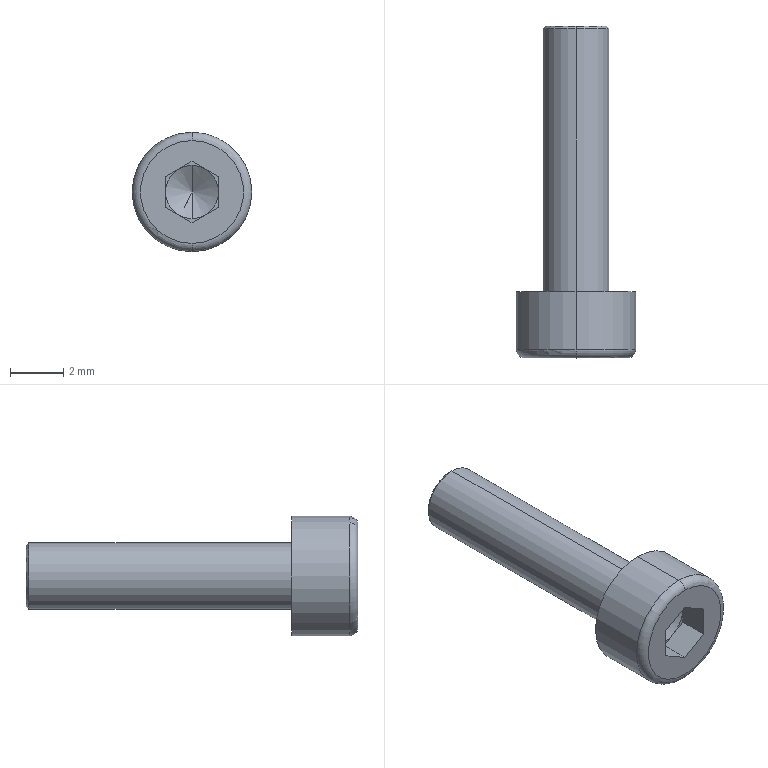Component | SolidWorks | hexagon socket head cap screws gb-10 | 1 solid | 25 faces | box 4.5 x 12.5 x 4.5 mm | volume 84 mm3 | plane 15 | cone 4 | cylinder 4 | torus 2 | commonest cylinder face diameters 2.5 x2 4.5 x2
build123d program:
from build123d import *

# Parameters (mm, degrees)
SKETCH1_R           = 2.25
BASEHEAD_DEPTH      = 2.5
SKETCH2_R           = 1.25
BASEBODY_DEPTH      = 10
HEXAGONSOCKET_DEPTH = 1.1
TOPFILLET_R         = 0.3125
CHAMFER1_SIZE       = 0.1


with BuildPart() as part:
    # Sketch1 → BaseHead (new body)
    with BuildSketch(Plane(origin=(0, 0, 0), x_dir=(0, 0, -1), z_dir=(1, 0, 0))):
        Circle(SKETCH1_R)
    extrude(amount=BASEHEAD_DEPTH)

    # Sketch2 → BaseBody (add)
    with BuildSketch(Plane(origin=(2.5, 0, 0), x_dir=(0, 0, -1), z_dir=(1, 0, 0))):
        Circle(SKETCH2_R)
    extrude(amount=BASEBODY_DEPTH)

    # Sketch3 → HexagonSocket (cut)
    with BuildSketch(Plane(origin=(0, 0, 0), x_dir=(0, 0, -1), z_dir=(1, 0, 0))):
        Polygon((1.155, 0), (0.5774, 1), (-0.5774, 1), (-1.155, 0), (-0.5774, -1), (0.5774, -1), align=None)
    extrude(amount=HEXAGONSOCKET_DEPTH, mode=Mode.SUBTRACT)

    # Sketch4 → Cut-Revolve1 (revolve, cut)
    with BuildSketch(Plane(origin=(-4.196, 0.75, 0), x_dir=(-1, 0, 0), z_dir=(0, 0, 1)), mode=Mode.PRIVATE) as cut_revolve1_sk:
        Polygon((-5.296, 1.75), (-5.873, 0.75), (-5.296, 0.75), align=None)
    revolve(cut_revolve1_sk.sketch.rotate(Axis((0.839, 0, 0), (-1, 0, 0)), 90), axis=Axis((0.839, 0, 0), (-1, 0, 0)), mode=Mode.SUBTRACT)

    # TopFillet
    topfillet_edges = [part.edges().sort_by_distance(p)[0] for p in [
        (0, 0, 2.25),
    ]]
    fillet(topfillet_edges, radius=TOPFILLET_R)

    # Chamfer1
    chamfer1_edges = [part.edges().sort_by_distance(p)[0] for p in [
        (12.5, 0, 1.25),
    ]]
    chamfer(chamfer1_edges, length=CHAMFER1_SIZE)


solid = part.part

# Placed as in the assembly
solid = solid.moved(Location((51.034, -16.994, 238.475), (0, 0, 90)))
STEP:
#1=CARTESIAN_POINT('',(2.009,-0.1769,9.343));
#2=VERTEX_POINT('',#1);
#3=CARTESIAN_POINT('',(2.009,-0.1769,9.434));
#4=VERTEX_POINT('',#3);
#5=CARTESIAN_POINT('',(2.009,-0.1769,9.389));
#6=DIRECTION('',(0.,1.,0.));
#7=DIRECTION('',(0.,0.,-1.));
#8=AXIS2_PLACEMENT_3D('',#5,#6,#7);
#9=CIRCLE('',#8,0.04528);
#10=EDGE_CURVE('',#2,#4,#9,.T.);
#11=ORIENTED_EDGE('',*,*,#10,.F.);
#12=CARTESIAN_POINT('',(2.009,-0.1809,9.34));
#13=VERTEX_POINT('',#12);
#14=CARTESIAN_POINT('',(2.009,-0.1769,9.343));
#15=DIRECTION('',(-0.,-0.7071,-0.7071));
#16=VECTOR('',#15,39.37);
#17=LINE('',#14,#16);
#18=EDGE_CURVE('',#2,#13,#17,.T.);
#19=ORIENTED_EDGE('',*,*,#18,.T.);
#20=CARTESIAN_POINT('',(2.009,-0.1809,9.438));
#21=VERTEX_POINT('',#20);
#22=CARTESIAN_POINT('',(2.009,-0.1809,9.389));
#23=DIRECTION('',(0.,-1.,0.));
#24=DIRECTION('',(0.,0.,-1.));
#25=AXIS2_PLACEMENT_3D('',#22,#23,#24);
#26=CIRCLE('',#25,0.04921);
#27=EDGE_CURVE('',#21,#13,#26,.T.);
#28=ORIENTED_EDGE('',*,*,#27,.F.);
#29=CARTESIAN_POINT('',(2.009,-0.1769,9.434));
#30=DIRECTION('',(0.,-0.7071,0.7071));
#31=VECTOR('',#30,39.37);
#32=LINE('',#29,#31);
#33=EDGE_CURVE('',#4,#21,#32,.T.);
#34=ORIENTED_EDGE('',*,*,#33,.F.);
#35=EDGE_LOOP('',(#11,#19,#28,#34));
#36=FACE_OUTER_BOUND('',#35,.T.);
#37=CARTESIAN_POINT('',(2.009,-0.1769,9.389));
#38=DIRECTION('',(0.,-1.,0.));
#39=DIRECTION('',(0.,0.,1.));
#40=AXIS2_PLACEMENT_3D('',#37,#38,#39);
#41=CONICAL_SURFACE('',#40,0.04528,0.7854);
#42=ADVANCED_FACE('',(#36),#41,.T.);
#43=CARTESIAN_POINT('',(2.009,-0.669,9.465));
#44=VERTEX_POINT('',#43);
#45=CARTESIAN_POINT('',(2.009,-0.669,9.312));
#46=VERTEX_POINT('',#45);
#47=CARTESIAN_POINT('',(2.009,-0.669,9.389));
#48=DIRECTION('',(0.,-1.,0.));
#49=DIRECTION('',(0.,0.,-1.));
#50=AXIS2_PLACEMENT_3D('',#47,#48,#49);
#51=CIRCLE('',#50,0.07628);
#52=EDGE_CURVE('',#44,#46,#51,.T.);
#53=ORIENTED_EDGE('',*,*,#52,.F.);
#54=CARTESIAN_POINT('',(2.009,-0.6567,9.477));
#55=VERTEX_POINT('',#54);
#56=CARTESIAN_POINT('',(2.009,-0.6567,9.465));
#57=DIRECTION('',(-1.,0.,-0.));
#58=DIRECTION('',(0.,0.,1.));
#59=AXIS2_PLACEMENT_3D('',#56,#57,#58);
#60=CIRCLE('',#59,0.0123);
#61=EDGE_CURVE('',#44,#55,#60,.T.);
#62=ORIENTED_EDGE('',*,*,#61,.T.);
#63=CARTESIAN_POINT('',(2.009,-0.6567,9.3));
#64=VERTEX_POINT('',#63);
#65=CARTESIAN_POINT('',(2.009,-0.6567,9.389));
#66=DIRECTION('',(0.,1.,0.));
#67=DIRECTION('',(0.,0.,-1.));
#68=AXIS2_PLACEMENT_3D('',#65,#66,#67);
#69=CIRCLE('',#68,0.08858);
#70=EDGE_CURVE('',#64,#55,#69,.T.);
#71=ORIENTED_EDGE('',*,*,#70,.F.);
#72=CARTESIAN_POINT('',(2.009,-0.6567,9.312));
#73=DIRECTION('',(1.,0.,0.));
#74=DIRECTION('',(0.,0.,-1.));
#75=AXIS2_PLACEMENT_3D('',#72,#73,#74);
#76=CIRCLE('',#75,0.0123);
#77=EDGE_CURVE('',#46,#64,#76,.T.);
#78=ORIENTED_EDGE('',*,*,#77,.F.);
#79=EDGE_LOOP('',(#53,#62,#71,#78));
#80=FACE_OUTER_BOUND('',#79,.T.);
#81=CARTESIAN_POINT('',(2.009,-0.6567,9.389));
#82=DIRECTION('',(0.,1.,0.));
#83=DIRECTION('',(0.,0.,-1.));
#84=AXIS2_PLACEMENT_3D('',#81,#82,#83);
#85=TOROIDAL_SURFACE('',#84,0.07628,0.0123);
#86=ADVANCED_FACE('',(#80),#85,.T.);
#87=CARTESIAN_POINT('',(2.009,-0.603,9.389));
#88=VERTEX_POINT('',#87);
#89=CARTESIAN_POINT('',(2.009,-0.6257,9.428));
#90=VERTEX_POINT('',#89);
#91=CARTESIAN_POINT('',(2.009,-0.6257,9.428));
#92=DIRECTION('',(0.,-0.5,0.866));
#93=VECTOR('',#92,39.37);
#94=LINE('',#91,#93);
#95=EDGE_CURVE('',#88,#90,#94,.T.);
#96=ORIENTED_EDGE('',*,*,#95,.F.);
#97=CARTESIAN_POINT('',(2.009,-0.6257,9.349));
#98=VERTEX_POINT('',#97);
#99=CARTESIAN_POINT('',(2.009,-0.6257,9.349));
#100=DIRECTION('',(-0.,-0.5,-0.866));
#101=VECTOR('',#100,39.37);
#102=LINE('',#99,#101);
#103=EDGE_CURVE('',#88,#98,#102,.T.);
#104=ORIENTED_EDGE('',*,*,#103,.T.);
#105=CARTESIAN_POINT('',(2.029,-0.6257,9.355));
#106=VERTEX_POINT('',#105);
#107=CARTESIAN_POINT('',(2.009,-0.6257,9.389));
#108=DIRECTION('',(0.,-1.,0.));
#109=DIRECTION('',(0.,0.,-1.));
#110=AXIS2_PLACEMENT_3D('',#107,#108,#109);
#111=CIRCLE('',#110,0.03937);
#112=EDGE_CURVE('',#98,#106,#111,.T.);
#113=ORIENTED_EDGE('',*,*,#112,.T.);
#114=CARTESIAN_POINT('',(2.049,-0.6257,9.389));
#115=VERTEX_POINT('',#114);
#116=CARTESIAN_POINT('',(2.009,-0.6257,9.389));
#117=DIRECTION('',(0.,-1.,0.));
#118=DIRECTION('',(0.,0.,-1.));
#119=AXIS2_PLACEMENT_3D('',#116,#117,#118);
#120=CIRCLE('',#119,0.03937);
#121=EDGE_CURVE('',#106,#115,#120,.T.);
#122=ORIENTED_EDGE('',*,*,#121,.T.);
#123=CARTESIAN_POINT('',(2.029,-0.6257,9.423));
#124=VERTEX_POINT('',#123);
#125=CARTESIAN_POINT('',(2.009,-0.6257,9.389));
#126=DIRECTION('',(0.,-1.,0.));
#127=DIRECTION('',(0.,0.,-1.));
#128=AXIS2_PLACEMENT_3D('',#125,#126,#127);
#129=CIRCLE('',#128,0.03937);
#130=EDGE_CURVE('',#115,#124,#129,.T.);
#131=ORIENTED_EDGE('',*,*,#130,.T.);
#132=CARTESIAN_POINT('',(2.009,-0.6257,9.389));
#133=DIRECTION('',(0.,-1.,0.));
#134=DIRECTION('',(0.,0.,-1.));
#135=AXIS2_PLACEMENT_3D('',#132,#133,#134);
#136=CIRCLE('',#135,0.03937);
#137=EDGE_CURVE('',#124,#90,#136,.T.);
#138=ORIENTED_EDGE('',*,*,#137,.T.);
#139=EDGE_LOOP('',(#96,#104,#113,#122,#131,#138));
#140=FACE_OUTER_BOUND('',#139,.T.);
#141=CARTESIAN_POINT('',(2.009,-0.6257,9.389));
#142=DIRECTION('',(0.,-1.,0.));
#143=DIRECTION('',(0.,0.,1.));
#144=AXIS2_PLACEMENT_3D('',#141,#142,#143);
#145=CONICAL_SURFACE('',#144,0.03937,1.047);
#146=ADVANCED_FACE('',(#140),#145,.F.);
#147=ORIENTED_EDGE('',*,*,#27,.T.);
#148=CARTESIAN_POINT('',(2.009,-0.5706,9.34));
#149=VERTEX_POINT('',#148);
#150=CARTESIAN_POINT('',(2.009,-0.1769,9.34));
#151=DIRECTION('',(0.,-1.,0.));
#152=VECTOR('',#151,39.37);
#153=LINE('',#150,#152);
#154=EDGE_CURVE('',#13,#149,#153,.T.);
#155=ORIENTED_EDGE('',*,*,#154,.T.);
#156=CARTESIAN_POINT('',(2.009,-0.5706,9.438));
#157=VERTEX_POINT('',#156);
#158=CARTESIAN_POINT('',(2.009,-0.5706,9.389));
#159=DIRECTION('',(0.,1.,0.));
#160=DIRECTION('',(0.,0.,-1.));
#161=AXIS2_PLACEMENT_3D('',#158,#159,#160);
#162=CIRCLE('',#161,0.04921);
#163=EDGE_CURVE('',#149,#157,#162,.T.);
#164=ORIENTED_EDGE('',*,*,#163,.T.);
#165=CARTESIAN_POINT('',(2.009,-0.1769,9.438));
#166=DIRECTION('',(0.,-1.,0.));
#167=VECTOR('',#166,39.37);
#168=LINE('',#165,#167);
#169=EDGE_CURVE('',#21,#157,#168,.T.);
#170=ORIENTED_EDGE('',*,*,#169,.F.);
#171=EDGE_LOOP('',(#147,#155,#164,#170));
#172=FACE_OUTER_BOUND('',#171,.T.);
#173=CARTESIAN_POINT('',(2.009,-0.1769,9.389));
#174=DIRECTION('',(0.,-1.,0.));
#175=DIRECTION('',(0.,0.,1.));
#176=AXIS2_PLACEMENT_3D('',#173,#174,#175);
#177=CYLINDRICAL_SURFACE('',#176,0.04921);
#178=ADVANCED_FACE('',(#172),#177,.T.);
#179=CARTESIAN_POINT('',(2.009,-0.5706,9.3));
#180=VERTEX_POINT('',#179);
#181=CARTESIAN_POINT('',(2.009,-0.5706,9.477));
#182=VERTEX_POINT('',#181);
#183=CARTESIAN_POINT('',(2.009,-0.5706,9.389));
#184=DIRECTION('',(0.,1.,0.));
#185=DIRECTION('',(0.,0.,-1.));
#186=AXIS2_PLACEMENT_3D('',#183,#184,#185);
#187=CIRCLE('',#186,0.08858);
#188=EDGE_CURVE('',#180,#182,#187,.T.);
#189=ORIENTED_EDGE('',*,*,#188,.F.);
#190=CARTESIAN_POINT('',(2.009,-0.5706,9.3));
#191=DIRECTION('',(0.,-1.,0.));
#192=VECTOR('',#191,39.37);
#193=LINE('',#190,#192);
#194=EDGE_CURVE('',#180,#64,#193,.T.);
#195=ORIENTED_EDGE('',*,*,#194,.T.);
#196=ORIENTED_EDGE('',*,*,#70,.T.);
#197=CARTESIAN_POINT('',(2.009,-0.5706,9.477));
#198=DIRECTION('',(0.,-1.,0.));
#199=VECTOR('',#198,39.37);
#200=LINE('',#197,#199);
#201=EDGE_CURVE('',#182,#55,#200,.T.);
#202=ORIENTED_EDGE('',*,*,#201,.F.);
#203=EDGE_LOOP('',(#189,#195,#196,#202));
#204=FACE_OUTER_BOUND('',#203,.T.);
#205=CARTESIAN_POINT('',(2.009,-0.5706,9.389));
#206=DIRECTION('',(0.,-1.,0.));
#207=DIRECTION('',(0.,0.,1.));
#208=AXIS2_PLACEMENT_3D('',#205,#206,#207);
#209=CYLINDRICAL_SURFACE('',#208,0.08858);
#210=ADVANCED_FACE('',(#204),#209,.T.);
#211=ORIENTED_EDGE('',*,*,#121,.F.);
#212=CARTESIAN_POINT('',(2.049,-0.6257,9.366));
#213=VERTEX_POINT('',#212);
#214=CARTESIAN_POINT('',(2.049,-0.6257,9.366));
#215=DIRECTION('',(-0.866,0.,-0.5));
#216=VECTOR('',#215,39.37);
#217=LINE('',#214,#216);
#218=EDGE_CURVE('',#213,#106,#217,.T.);
#219=ORIENTED_EDGE('',*,*,#218,.F.);
#220=CARTESIAN_POINT('',(2.049,-0.6257,9.411));
#221=DIRECTION('',(-0.,0.,-1.));
#222=VECTOR('',#221,39.37);
#223=LINE('',#220,#222);
#224=EDGE_CURVE('',#115,#213,#223,.T.);
#225=ORIENTED_EDGE('',*,*,#224,.F.);
#226=EDGE_LOOP('',(#211,#219,#225));
#227=FACE_OUTER_BOUND('',#226,.T.);
#228=CARTESIAN_POINT('',(2.009,-0.6257,9.343));
#229=DIRECTION('',(0.,1.,0.));
#230=DIRECTION('',(0.,0.,-1.));
#231=AXIS2_PLACEMENT_3D('',#228,#229,#230);
#232=PLANE('',#231);
#233=ADVANCED_FACE('',(#227),#232,.F.);
#234=ORIENTED_EDGE('',*,*,#130,.F.);
#235=CARTESIAN_POINT('',(2.049,-0.6257,9.411));
#236=VERTEX_POINT('',#235);
#237=CARTESIAN_POINT('',(2.049,-0.6257,9.411));
#238=DIRECTION('',(-0.,0.,-1.));
#239=VECTOR('',#238,39.37);
#240=LINE('',#237,#239);
#241=EDGE_CURVE('',#236,#115,#240,.T.);
#242=ORIENTED_EDGE('',*,*,#241,.F.);
#243=CARTESIAN_POINT('',(2.009,-0.6257,9.434));
#244=DIRECTION('',(0.866,0.,-0.5));
#245=VECTOR('',#244,39.37);
#246=LINE('',#243,#245);
#247=EDGE_CURVE('',#124,#236,#246,.T.);
#248=ORIENTED_EDGE('',*,*,#247,.F.);
#249=EDGE_LOOP('',(#234,#242,#248));
#250=FACE_OUTER_BOUND('',#249,.T.);
#251=CARTESIAN_POINT('',(2.009,-0.6257,9.343));
#252=DIRECTION('',(0.,1.,0.));
#253=DIRECTION('',(0.,0.,-1.));
#254=AXIS2_PLACEMENT_3D('',#251,#252,#253);
#255=PLANE('',#254);
#256=ADVANCED_FACE('',(#250),#255,.F.);
#257=ORIENTED_EDGE('',*,*,#137,.F.);
#258=CARTESIAN_POINT('',(2.009,-0.6257,9.434));
#259=VERTEX_POINT('',#258);
#260=CARTESIAN_POINT('',(2.009,-0.6257,9.434));
#261=DIRECTION('',(0.866,0.,-0.5));
#262=VECTOR('',#261,39.37);
#263=LINE('',#260,#262);
#264=EDGE_CURVE('',#259,#124,#263,.T.);
#265=ORIENTED_EDGE('',*,*,#264,.F.);
#266=CARTESIAN_POINT('',(1.99,-0.6257,9.423));
#267=VERTEX_POINT('',#266);
#268=CARTESIAN_POINT('',(1.97,-0.6257,9.411));
#269=DIRECTION('',(0.866,0.,0.5));
#270=VECTOR('',#269,39.37);
#271=LINE('',#268,#270);
#272=EDGE_CURVE('',#267,#259,#271,.T.);
#273=ORIENTED_EDGE('',*,*,#272,.F.);
#274=CARTESIAN_POINT('',(2.009,-0.6257,9.389));
#275=DIRECTION('',(0.,-1.,0.));
#276=DIRECTION('',(0.,0.,-1.));
#277=AXIS2_PLACEMENT_3D('',#274,#275,#276);
#278=CIRCLE('',#277,0.03937);
#279=EDGE_CURVE('',#90,#267,#278,.T.);
#280=ORIENTED_EDGE('',*,*,#279,.F.);
#281=EDGE_LOOP('',(#257,#265,#273,#280));
#282=FACE_OUTER_BOUND('',#281,.T.);
#283=CARTESIAN_POINT('',(2.009,-0.6257,9.343));
#284=DIRECTION('',(0.,1.,0.));
#285=DIRECTION('',(0.,0.,-1.));
#286=AXIS2_PLACEMENT_3D('',#283,#284,#285);
#287=PLANE('',#286);
#288=ADVANCED_FACE('',(#282),#287,.F.);
#289=CARTESIAN_POINT('',(1.97,-0.6257,9.389));
#290=VERTEX_POINT('',#289);
#291=CARTESIAN_POINT('',(2.009,-0.6257,9.389));
#292=DIRECTION('',(0.,-1.,0.));
#293=DIRECTION('',(0.,0.,-1.));
#294=AXIS2_PLACEMENT_3D('',#291,#292,#293);
#295=CIRCLE('',#294,0.03937);
#296=EDGE_CURVE('',#267,#290,#295,.T.);
#297=ORIENTED_EDGE('',*,*,#296,.F.);
#298=CARTESIAN_POINT('',(1.97,-0.6257,9.411));
#299=VERTEX_POINT('',#298);
#300=CARTESIAN_POINT('',(1.97,-0.6257,9.411));
#301=DIRECTION('',(0.866,0.,0.5));
#302=VECTOR('',#301,39.37);
#303=LINE('',#300,#302);
#304=EDGE_CURVE('',#299,#267,#303,.T.);
#305=ORIENTED_EDGE('',*,*,#304,.F.);
#306=CARTESIAN_POINT('',(1.97,-0.6257,9.366));
#307=DIRECTION('',(0.,0.,1.));
#308=VECTOR('',#307,39.37);
#309=LINE('',#306,#308);
#310=EDGE_CURVE('',#290,#299,#309,.T.);
#311=ORIENTED_EDGE('',*,*,#310,.F.);
#312=EDGE_LOOP('',(#297,#305,#311));
#313=FACE_OUTER_BOUND('',#312,.T.);
#314=CARTESIAN_POINT('',(2.009,-0.6257,9.343));
#315=DIRECTION('',(0.,1.,0.));
#316=DIRECTION('',(0.,0.,-1.));
#317=AXIS2_PLACEMENT_3D('',#314,#315,#316);
#318=PLANE('',#317);
#319=ADVANCED_FACE('',(#313),#318,.F.);
#320=CARTESIAN_POINT('',(1.99,-0.6257,9.355));
#321=VERTEX_POINT('',#320);
#322=CARTESIAN_POINT('',(2.009,-0.6257,9.389));
#323=DIRECTION('',(0.,1.,0.));
#324=DIRECTION('',(0.,0.,-1.));
#325=AXIS2_PLACEMENT_3D('',#322,#323,#324);
#326=CIRCLE('',#325,0.03937);
#327=EDGE_CURVE('',#321,#290,#326,.T.);
#328=ORIENTED_EDGE('',*,*,#327,.T.);
#329=CARTESIAN_POINT('',(1.97,-0.6257,9.366));
#330=VERTEX_POINT('',#329);
#331=CARTESIAN_POINT('',(1.97,-0.6257,9.366));
#332=DIRECTION('',(0.,0.,1.));
#333=VECTOR('',#332,39.37);
#334=LINE('',#331,#333);
#335=EDGE_CURVE('',#330,#290,#334,.T.);
#336=ORIENTED_EDGE('',*,*,#335,.F.);
#337=CARTESIAN_POINT('',(2.009,-0.6257,9.343));
#338=DIRECTION('',(-0.866,0.,0.5));
#339=VECTOR('',#338,39.37);
#340=LINE('',#337,#339);
#341=EDGE_CURVE('',#321,#330,#340,.T.);
#342=ORIENTED_EDGE('',*,*,#341,.F.);
#343=EDGE_LOOP('',(#328,#336,#342));
#344=FACE_OUTER_BOUND('',#343,.T.);
#345=CARTESIAN_POINT('',(2.009,-0.6257,9.343));
#346=DIRECTION('',(0.,1.,0.));
#347=DIRECTION('',(0.,0.,-1.));
#348=AXIS2_PLACEMENT_3D('',#345,#346,#347);
#349=PLANE('',#348);
#350=ADVANCED_FACE('',(#344),#349,.F.);
#351=CARTESIAN_POINT('',(2.009,-0.6257,9.389));
#352=DIRECTION('',(0.,-1.,0.));
#353=DIRECTION('',(0.,0.,-1.));
#354=AXIS2_PLACEMENT_3D('',#351,#352,#353);
#355=CIRCLE('',#354,0.03937);
#356=EDGE_CURVE('',#321,#98,#355,.T.);
#357=ORIENTED_EDGE('',*,*,#356,.F.);
#358=CARTESIAN_POINT('',(2.009,-0.6257,9.343));
#359=VERTEX_POINT('',#358);
#360=CARTESIAN_POINT('',(2.009,-0.6257,9.343));
#361=DIRECTION('',(-0.866,0.,0.5));
#362=VECTOR('',#361,39.37);
#363=LINE('',#360,#362);
#364=EDGE_CURVE('',#359,#321,#363,.T.);
#365=ORIENTED_EDGE('',*,*,#364,.F.);
#366=CARTESIAN_POINT('',(2.049,-0.6257,9.366));
#367=DIRECTION('',(-0.866,0.,-0.5));
#368=VECTOR('',#367,39.37);
#369=LINE('',#366,#368);
#370=EDGE_CURVE('',#106,#359,#369,.T.);
#371=ORIENTED_EDGE('',*,*,#370,.F.);
#372=ORIENTED_EDGE('',*,*,#112,.F.);
#373=EDGE_LOOP('',(#357,#365,#371,#372));
#374=FACE_OUTER_BOUND('',#373,.T.);
#375=CARTESIAN_POINT('',(2.009,-0.6257,9.343));
#376=DIRECTION('',(0.,1.,0.));
#377=DIRECTION('',(0.,0.,-1.));
#378=AXIS2_PLACEMENT_3D('',#375,#376,#377);
#379=PLANE('',#378);
#380=ADVANCED_FACE('',(#374),#379,.F.);
#381=CARTESIAN_POINT('',(2.009,-0.669,9.389));
#382=DIRECTION('',(0.,-1.,0.));
#383=DIRECTION('',(0.,0.,-1.));
#384=AXIS2_PLACEMENT_3D('',#381,#382,#383);
#385=CIRCLE('',#384,0.07628);
#386=EDGE_CURVE('',#46,#44,#385,.T.);
#387=ORIENTED_EDGE('',*,*,#386,.T.);
#388=ORIENTED_EDGE('',*,*,#52,.T.);
#389=EDGE_LOOP('',(#387,#388));
#390=FACE_OUTER_BOUND('',#389,.T.);
#391=CARTESIAN_POINT('',(2.049,-0.669,9.366));
#392=VERTEX_POINT('',#391);
#393=CARTESIAN_POINT('',(2.009,-0.669,9.343));
#394=VERTEX_POINT('',#393);
#395=CARTESIAN_POINT('',(2.049,-0.669,9.366));
#396=DIRECTION('',(-0.866,0.,-0.5));
#397=VECTOR('',#396,39.37);
#398=LINE('',#395,#397);
#399=EDGE_CURVE('',#392,#394,#398,.T.);
#400=ORIENTED_EDGE('',*,*,#399,.T.);
#401=CARTESIAN_POINT('',(1.97,-0.669,9.366));
#402=VERTEX_POINT('',#401);
#403=CARTESIAN_POINT('',(2.009,-0.669,9.343));
#404=DIRECTION('',(-0.866,0.,0.5));
#405=VECTOR('',#404,39.37);
#406=LINE('',#403,#405);
#407=EDGE_CURVE('',#394,#402,#406,.T.);
#408=ORIENTED_EDGE('',*,*,#407,.T.);
#409=CARTESIAN_POINT('',(1.97,-0.669,9.411));
#410=VERTEX_POINT('',#409);
#411=CARTESIAN_POINT('',(1.97,-0.669,9.366));
#412=DIRECTION('',(0.,0.,1.));
#413=VECTOR('',#412,39.37);
#414=LINE('',#411,#413);
#415=EDGE_CURVE('',#402,#410,#414,.T.);
#416=ORIENTED_EDGE('',*,*,#415,.T.);
#417=CARTESIAN_POINT('',(2.009,-0.669,9.434));
#418=VERTEX_POINT('',#417);
#419=CARTESIAN_POINT('',(1.97,-0.669,9.411));
#420=DIRECTION('',(0.866,0.,0.5));
#421=VECTOR('',#420,39.37);
#422=LINE('',#419,#421);
#423=EDGE_CURVE('',#410,#418,#422,.T.);
#424=ORIENTED_EDGE('',*,*,#423,.T.);
#425=CARTESIAN_POINT('',(2.049,-0.669,9.411));
#426=VERTEX_POINT('',#425);
#427=CARTESIAN_POINT('',(2.009,-0.669,9.434));
#428=DIRECTION('',(0.866,0.,-0.5));
#429=VECTOR('',#428,39.37);
#430=LINE('',#427,#429);
#431=EDGE_CURVE('',#418,#426,#430,.T.);
#432=ORIENTED_EDGE('',*,*,#431,.T.);
#433=CARTESIAN_POINT('',(2.049,-0.669,9.411));
#434=DIRECTION('',(-0.,0.,-1.));
#435=VECTOR('',#434,39.37);
#436=LINE('',#433,#435);
#437=EDGE_CURVE('',#426,#392,#436,.T.);
#438=ORIENTED_EDGE('',*,*,#437,.T.);
#439=EDGE_LOOP('',(#400,#408,#416,#424,#432,#438));
#440=FACE_BOUND('',#439,.T.);
#441=CARTESIAN_POINT('',(2.009,-0.669,9.389));
#442=DIRECTION('',(0.,1.,0.));
#443=DIRECTION('',(0.,0.,-1.));
#444=AXIS2_PLACEMENT_3D('',#441,#442,#443);
#445=PLANE('',#444);
#446=ADVANCED_FACE('',(#390,#440),#445,.F.);
#447=CARTESIAN_POINT('',(2.009,-0.5706,9.389));
#448=DIRECTION('',(0.,1.,0.));
#449=DIRECTION('',(0.,0.,-1.));
#450=AXIS2_PLACEMENT_3D('',#447,#448,#449);
#451=CIRCLE('',#450,0.08858);
#452=EDGE_CURVE('',#182,#180,#451,.T.);
#453=ORIENTED_EDGE('',*,*,#452,.T.);
#454=ORIENTED_EDGE('',*,*,#188,.T.);
#455=EDGE_LOOP('',(#453,#454));
#456=FACE_OUTER_BOUND('',#455,.T.);
#457=CARTESIAN_POINT('',(2.009,-0.5706,9.389));
#458=DIRECTION('',(0.,1.,0.));
#459=DIRECTION('',(0.,0.,-1.));
#460=AXIS2_PLACEMENT_3D('',#457,#458,#459);
#461=CIRCLE('',#460,0.04921);
#462=EDGE_CURVE('',#157,#149,#461,.T.);
#463=ORIENTED_EDGE('',*,*,#462,.F.);
#464=ORIENTED_EDGE('',*,*,#163,.F.);
#465=EDGE_LOOP('',(#463,#464));
#466=FACE_BOUND('',#465,.T.);
#467=CARTESIAN_POINT('',(2.009,-0.5706,9.389));
#468=DIRECTION('',(0.,1.,0.));
#469=DIRECTION('',(0.,0.,-1.));
#470=AXIS2_PLACEMENT_3D('',#467,#468,#469);
#471=PLANE('',#470);
#472=ADVANCED_FACE('',(#456,#466),#471,.T.);
#473=ORIENTED_EDGE('',*,*,#194,.F.);
#474=ORIENTED_EDGE('',*,*,#452,.F.);
#475=ORIENTED_EDGE('',*,*,#201,.T.);
#476=CARTESIAN_POINT('',(2.009,-0.6567,9.389));
#477=DIRECTION('',(0.,1.,0.));
#478=DIRECTION('',(0.,0.,-1.));
#479=AXIS2_PLACEMENT_3D('',#476,#477,#478);
#480=CIRCLE('',#479,0.08858);
#481=EDGE_CURVE('',#55,#64,#480,.T.);
#482=ORIENTED_EDGE('',*,*,#481,.T.);
#483=EDGE_LOOP('',(#473,#474,#475,#482));
#484=FACE_OUTER_BOUND('',#483,.T.);
#485=CARTESIAN_POINT('',(2.009,-0.5706,9.389));
#486=DIRECTION('',(0.,-1.,0.));
#487=DIRECTION('',(0.,0.,1.));
#488=AXIS2_PLACEMENT_3D('',#485,#486,#487);
#489=CYLINDRICAL_SURFACE('',#488,0.08858);
#490=ADVANCED_FACE('',(#484),#489,.T.);
#491=ORIENTED_EDGE('',*,*,#154,.F.);
#492=CARTESIAN_POINT('',(2.009,-0.1809,9.389));
#493=DIRECTION('',(0.,-1.,0.));
#494=DIRECTION('',(0.,0.,-1.));
#495=AXIS2_PLACEMENT_3D('',#492,#493,#494);
#496=CIRCLE('',#495,0.04921);
#497=EDGE_CURVE('',#13,#21,#496,.T.);
#498=ORIENTED_EDGE('',*,*,#497,.T.);
#499=ORIENTED_EDGE('',*,*,#169,.T.);
#500=ORIENTED_EDGE('',*,*,#462,.T.);
#501=EDGE_LOOP('',(#491,#498,#499,#500));
#502=FACE_OUTER_BOUND('',#501,.T.);
#503=CARTESIAN_POINT('',(2.009,-0.1769,9.389));
#504=DIRECTION('',(0.,-1.,0.));
#505=DIRECTION('',(0.,0.,1.));
#506=AXIS2_PLACEMENT_3D('',#503,#504,#505);
#507=CYLINDRICAL_SURFACE('',#506,0.04921);
#508=ADVANCED_FACE('',(#502),#507,.T.);
#509=CARTESIAN_POINT('',(2.009,-0.1769,9.389));
#510=DIRECTION('',(0.,1.,0.));
#511=DIRECTION('',(0.,0.,-1.));
#512=AXIS2_PLACEMENT_3D('',#509,#510,#511);
#513=CIRCLE('',#512,0.04528);
#514=EDGE_CURVE('',#4,#2,#513,.T.);
#515=ORIENTED_EDGE('',*,*,#514,.T.);
#516=ORIENTED_EDGE('',*,*,#10,.T.);
#517=EDGE_LOOP('',(#515,#516));
#518=FACE_OUTER_BOUND('',#517,.T.);
#519=CARTESIAN_POINT('',(2.009,-0.1769,9.389));
#520=DIRECTION('',(0.,1.,0.));
#521=DIRECTION('',(0.,0.,-1.));
#522=AXIS2_PLACEMENT_3D('',#519,#520,#521);
#523=PLANE('',#522);
#524=ADVANCED_FACE('',(#518),#523,.T.);
#525=ORIENTED_EDGE('',*,*,#399,.F.);
#526=CARTESIAN_POINT('',(2.049,-0.6257,9.366));
#527=DIRECTION('',(0.,-1.,0.));
#528=VECTOR('',#527,39.37);
#529=LINE('',#526,#528);
#530=EDGE_CURVE('',#213,#392,#529,.T.);
#531=ORIENTED_EDGE('',*,*,#530,.F.);
#532=ORIENTED_EDGE('',*,*,#218,.T.);
#533=ORIENTED_EDGE('',*,*,#370,.T.);
#534=CARTESIAN_POINT('',(2.009,-0.6257,9.343));
#535=DIRECTION('',(0.,-1.,0.));
#536=VECTOR('',#535,39.37);
#537=LINE('',#534,#536);
#538=EDGE_CURVE('',#359,#394,#537,.T.);
#539=ORIENTED_EDGE('',*,*,#538,.T.);
#540=EDGE_LOOP('',(#525,#531,#532,#533,#539));
#541=FACE_OUTER_BOUND('',#540,.T.);
#542=CARTESIAN_POINT('',(2.049,-0.6257,9.366));
#543=DIRECTION('',(-0.5,0.,0.866));
#544=DIRECTION('',(0.866,0.,0.5));
#545=AXIS2_PLACEMENT_3D('',#542,#543,#544);
#546=PLANE('',#545);
#547=ADVANCED_FACE('',(#541),#546,.T.);
#548=ORIENTED_EDGE('',*,*,#407,.F.);
#549=ORIENTED_EDGE('',*,*,#538,.F.);
#550=ORIENTED_EDGE('',*,*,#364,.T.);
#551=ORIENTED_EDGE('',*,*,#341,.T.);
#552=CARTESIAN_POINT('',(1.97,-0.6257,9.366));
#553=DIRECTION('',(0.,-1.,0.));
#554=VECTOR('',#553,39.37);
#555=LINE('',#552,#554);
#556=EDGE_CURVE('',#330,#402,#555,.T.);
#557=ORIENTED_EDGE('',*,*,#556,.T.);
#558=EDGE_LOOP('',(#548,#549,#550,#551,#557));
#559=FACE_OUTER_BOUND('',#558,.T.);
#560=CARTESIAN_POINT('',(2.009,-0.6257,9.343));
#561=DIRECTION('',(0.5,0.,0.866));
#562=DIRECTION('',(0.866,0.,-0.5));
#563=AXIS2_PLACEMENT_3D('',#560,#561,#562);
#564=PLANE('',#563);
#565=ADVANCED_FACE('',(#559),#564,.T.);
#566=ORIENTED_EDGE('',*,*,#415,.F.);
#567=ORIENTED_EDGE('',*,*,#556,.F.);
#568=ORIENTED_EDGE('',*,*,#335,.T.);
#569=ORIENTED_EDGE('',*,*,#310,.T.);
#570=CARTESIAN_POINT('',(1.97,-0.6257,9.411));
#571=DIRECTION('',(0.,-1.,0.));
#572=VECTOR('',#571,39.37);
#573=LINE('',#570,#572);
#574=EDGE_CURVE('',#299,#410,#573,.T.);
#575=ORIENTED_EDGE('',*,*,#574,.T.);
#576=EDGE_LOOP('',(#566,#567,#568,#569,#575));
#577=FACE_OUTER_BOUND('',#576,.T.);
#578=CARTESIAN_POINT('',(1.97,-0.6257,9.366));
#579=DIRECTION('',(1.,0.,0.));
#580=DIRECTION('',(0.,0.,-1.));
#581=AXIS2_PLACEMENT_3D('',#578,#579,#580);
#582=PLANE('',#581);
#583=ADVANCED_FACE('',(#577),#582,.T.);
#584=ORIENTED_EDGE('',*,*,#423,.F.);
#585=ORIENTED_EDGE('',*,*,#574,.F.);
#586=ORIENTED_EDGE('',*,*,#304,.T.);
#587=ORIENTED_EDGE('',*,*,#272,.T.);
#588=CARTESIAN_POINT('',(2.009,-0.6257,9.434));
#589=DIRECTION('',(0.,-1.,0.));
#590=VECTOR('',#589,39.37);
#591=LINE('',#588,#590);
#592=EDGE_CURVE('',#259,#418,#591,.T.);
#593=ORIENTED_EDGE('',*,*,#592,.T.);
#594=EDGE_LOOP('',(#584,#585,#586,#587,#593));
#595=FACE_OUTER_BOUND('',#594,.T.);
#596=CARTESIAN_POINT('',(1.97,-0.6257,9.411));
#597=DIRECTION('',(0.5,0.,-0.866));
#598=DIRECTION('',(-0.866,0.,-0.5));
#599=AXIS2_PLACEMENT_3D('',#596,#597,#598);
#600=PLANE('',#599);
#601=ADVANCED_FACE('',(#595),#600,.T.);
#602=ORIENTED_EDGE('',*,*,#431,.F.);
#603=ORIENTED_EDGE('',*,*,#592,.F.);
#604=ORIENTED_EDGE('',*,*,#264,.T.);
#605=ORIENTED_EDGE('',*,*,#247,.T.);
#606=CARTESIAN_POINT('',(2.049,-0.6257,9.411));
#607=DIRECTION('',(0.,-1.,0.));
#608=VECTOR('',#607,39.37);
#609=LINE('',#606,#608);
#610=EDGE_CURVE('',#236,#426,#609,.T.);
#611=ORIENTED_EDGE('',*,*,#610,.T.);
#612=EDGE_LOOP('',(#602,#603,#604,#605,#611));
#613=FACE_OUTER_BOUND('',#612,.T.);
#614=CARTESIAN_POINT('',(2.009,-0.6257,9.434));
#615=DIRECTION('',(-0.5,0.,-0.866));
#616=DIRECTION('',(-0.866,0.,0.5));
#617=AXIS2_PLACEMENT_3D('',#614,#615,#616);
#618=PLANE('',#617);
#619=ADVANCED_FACE('',(#613),#618,.T.);
#620=ORIENTED_EDGE('',*,*,#437,.F.);
#621=ORIENTED_EDGE('',*,*,#610,.F.);
#622=ORIENTED_EDGE('',*,*,#241,.T.);
#623=ORIENTED_EDGE('',*,*,#224,.T.);
#624=ORIENTED_EDGE('',*,*,#530,.T.);
#625=EDGE_LOOP('',(#620,#621,#622,#623,#624));
#626=FACE_OUTER_BOUND('',#625,.T.);
#627=CARTESIAN_POINT('',(2.049,-0.6257,9.411));
#628=DIRECTION('',(-1.,0.,0.));
#629=DIRECTION('',(0.,0.,1.));
#630=AXIS2_PLACEMENT_3D('',#627,#628,#629);
#631=PLANE('',#630);
#632=ADVANCED_FACE('',(#626),#631,.T.);
#633=ORIENTED_EDGE('',*,*,#103,.F.);
#634=ORIENTED_EDGE('',*,*,#95,.T.);
#635=ORIENTED_EDGE('',*,*,#279,.T.);
#636=ORIENTED_EDGE('',*,*,#296,.T.);
#637=ORIENTED_EDGE('',*,*,#327,.F.);
#638=ORIENTED_EDGE('',*,*,#356,.T.);
#639=EDGE_LOOP('',(#633,#634,#635,#636,#637,#638));
#640=FACE_OUTER_BOUND('',#639,.T.);
#641=CARTESIAN_POINT('',(2.009,-0.6257,9.389));
#642=DIRECTION('',(0.,-1.,0.));
#643=DIRECTION('',(0.,0.,1.));
#644=AXIS2_PLACEMENT_3D('',#641,#642,#643);
#645=CONICAL_SURFACE('',#644,0.03937,1.047);
#646=ADVANCED_FACE('',(#640),#645,.F.);
#647=ORIENTED_EDGE('',*,*,#61,.F.);
#648=ORIENTED_EDGE('',*,*,#386,.F.);
#649=ORIENTED_EDGE('',*,*,#77,.T.);
#650=ORIENTED_EDGE('',*,*,#481,.F.);
#651=EDGE_LOOP('',(#647,#648,#649,#650));
#652=FACE_OUTER_BOUND('',#651,.T.);
#653=CARTESIAN_POINT('',(2.009,-0.6567,9.389));
#654=DIRECTION('',(0.,1.,0.));
#655=DIRECTION('',(0.,0.,-1.));
#656=AXIS2_PLACEMENT_3D('',#653,#654,#655);
#657=TOROIDAL_SURFACE('',#656,0.07628,0.0123);
#658=ADVANCED_FACE('',(#652),#657,.T.);
#659=ORIENTED_EDGE('',*,*,#18,.F.);
#660=ORIENTED_EDGE('',*,*,#514,.F.);
#661=ORIENTED_EDGE('',*,*,#33,.T.);
#662=ORIENTED_EDGE('',*,*,#497,.F.);
#663=EDGE_LOOP('',(#659,#660,#661,#662));
#664=FACE_OUTER_BOUND('',#663,.T.);
#665=CARTESIAN_POINT('',(2.009,-0.1769,9.389));
#666=DIRECTION('',(0.,-1.,0.));
#667=DIRECTION('',(0.,0.,1.));
#668=AXIS2_PLACEMENT_3D('',#665,#666,#667);
#669=CONICAL_SURFACE('',#668,0.04528,0.7854);
#670=ADVANCED_FACE('',(#664),#669,.T.);
#671=CLOSED_SHELL('',(#42,#86,#146,#178,#210,#233,#256,#288,#319,#350,#380,#446,#472,#490,#508,#524,#547,#565,#583,#601,#619,#632,#646,#658,#670));
#672=MANIFOLD_SOLID_BREP('',#671);
#673=CARTESIAN_POINT('',(0.,0.,0.));
#674=DIRECTION('',(0.,0.,1.));
#675=DIRECTION('',(1.,0.,0.));
#676=AXIS2_PLACEMENT_3D('',#673,#674,#675);
#677=(LENGTH_UNIT()NAMED_UNIT(*)SI_UNIT($,.METRE.));
#678=LENGTH_MEASURE_WITH_UNIT(LENGTH_MEASURE(0.0254),#677);
#679=DIMENSIONAL_EXPONENTS(1.,0.,0.,0.,0.,0.,0.);
#680=(CONVERSION_BASED_UNIT('',#678)LENGTH_UNIT()NAMED_UNIT(#679));
#681=UNCERTAINTY_MEASURE_WITH_UNIT(LENGTH_MEASURE(0.00001),#680,'','');
#682=(NAMED_UNIT(*)PLANE_ANGLE_UNIT()SI_UNIT($,.RADIAN.));
#683=(NAMED_UNIT(*)SI_UNIT($,.STERADIAN.)SOLID_ANGLE_UNIT());
#684=(GEOMETRIC_REPRESENTATION_CONTEXT(3)GLOBAL_UNCERTAINTY_ASSIGNED_CONTEXT((#681))GLOBAL_UNIT_ASSIGNED_CONTEXT((#680,#682,#683))REPRESENTATION_CONTEXT('',''));
#685=ADVANCED_BREP_SHAPE_REPRESENTATION('',(#672,#676),#684);
#686=COLOUR_RGB('',0.7922,0.8196,0.9333);
#687=FILL_AREA_STYLE_COLOUR('',#686);
#688=FILL_AREA_STYLE('',(#687));
#689=SURFACE_STYLE_FILL_AREA(#688);
#690=SURFACE_SIDE_STYLE('',(#689));
#691=SURFACE_STYLE_USAGE(.BOTH.,#690);
#692=PRESENTATION_STYLE_ASSIGNMENT((#691));
#693=STYLED_ITEM('',(#692),#672);
#694=PRESENTATION_LAYER_ASSIGNMENT('','',(#693));
#695=(LENGTH_UNIT()NAMED_UNIT(*)SI_UNIT($,.METRE.));
#696=LENGTH_MEASURE_WITH_UNIT(LENGTH_MEASURE(0.0254),#695);
#697=DIMENSIONAL_EXPONENTS(1.,0.,0.,0.,0.,0.,0.);
#698=(CONVERSION_BASED_UNIT('',#696)LENGTH_UNIT()NAMED_UNIT(#697));
#699=UNCERTAINTY_MEASURE_WITH_UNIT(LENGTH_MEASURE(0.00001),#698,'','');
#700=(NAMED_UNIT(*)PLANE_ANGLE_UNIT()SI_UNIT($,.RADIAN.));
#701=(NAMED_UNIT(*)SI_UNIT($,.STERADIAN.)SOLID_ANGLE_UNIT());
#702=(GEOMETRIC_REPRESENTATION_CONTEXT(3)GLOBAL_UNCERTAINTY_ASSIGNED_CONTEXT((#699))GLOBAL_UNIT_ASSIGNED_CONTEXT((#698,#700,#701))REPRESENTATION_CONTEXT('',''));
#703=MECHANICAL_DESIGN_GEOMETRIC_PRESENTATION_REPRESENTATION('',(#693),#702);